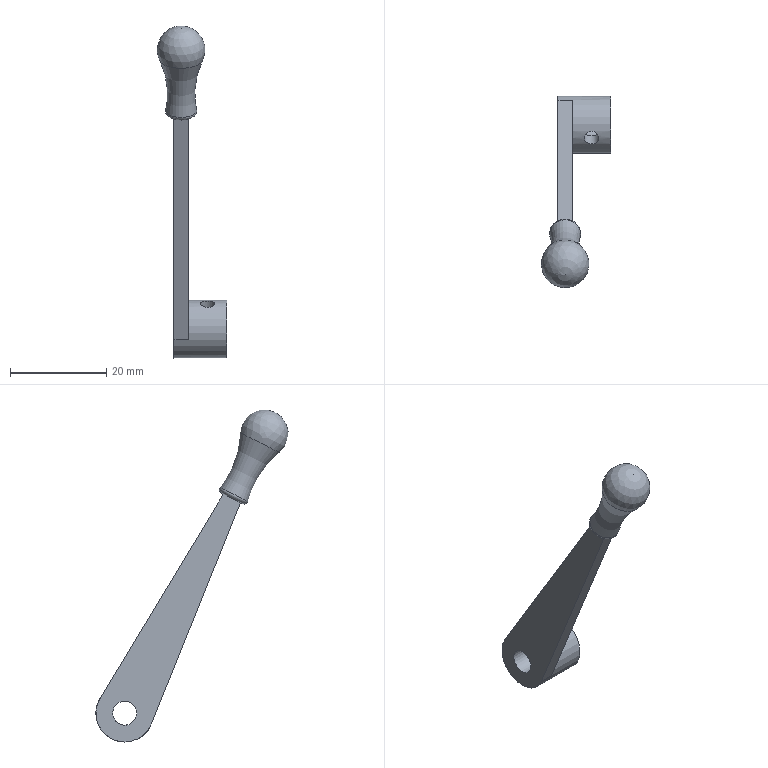Component | NX | 23A__27 | 1 solid | 16 faces | volume 2864 mm3 | plane 9 | cylinder 4 | torus 2 | sphere 1 | commonest cylinder face diameters 3 x2 12 x1 5 x1